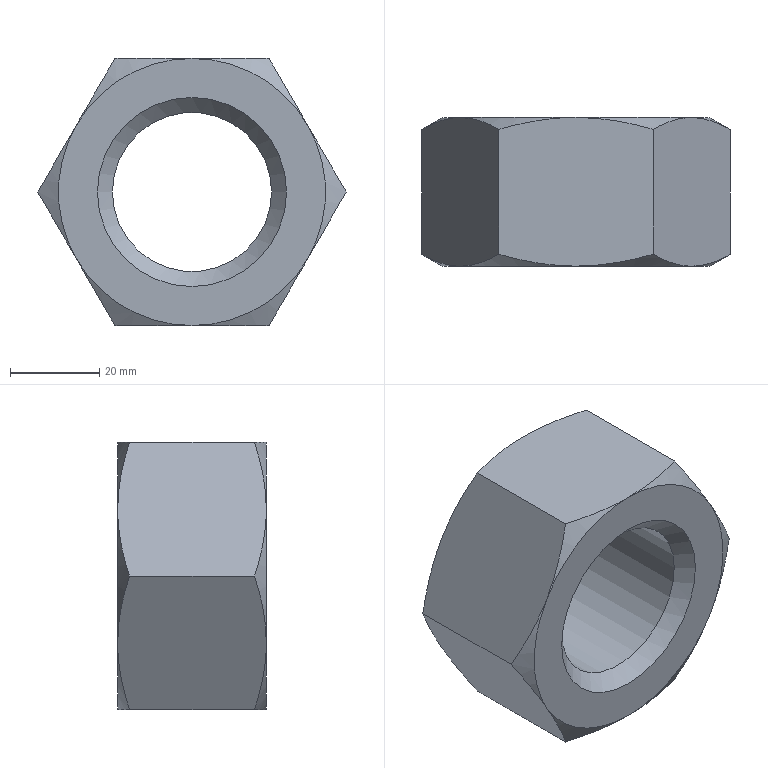Component | NX | GB-T6170_F-2000_M39X4 | 1 solid | 23 faces | volume 68776 mm3 | cone 14 | plane 8 | cylinder 1 | commonest cylinder face diameters 35.752 x1